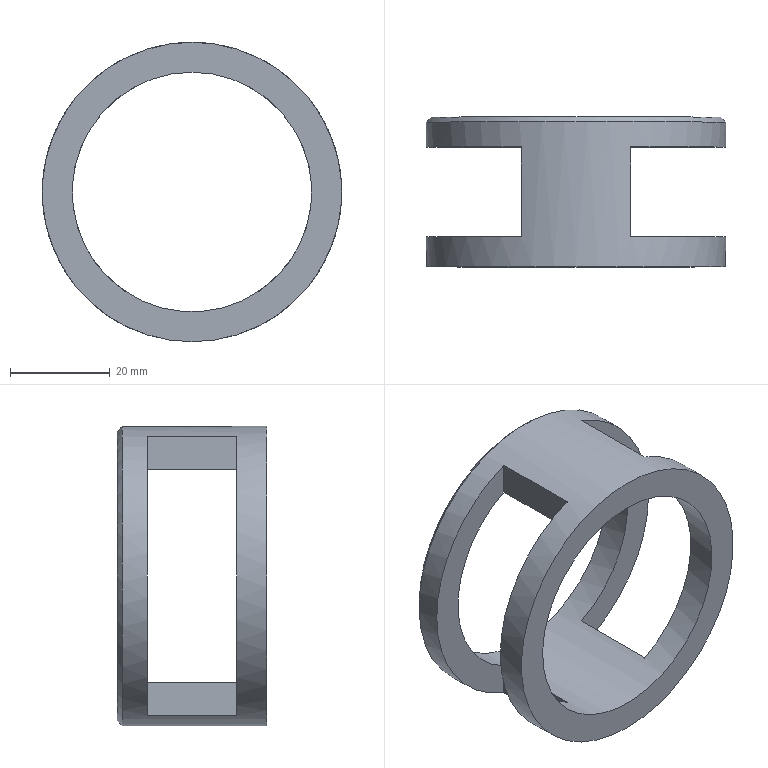Component | NX | BUSHING | 1 solid | 13 faces | box 60 x 30 x 60 mm | volume 17018 mm3 | plane 10 | cylinder 2 | cone 1 | commonest cylinder face diameters 60 x1 48 x1
STEP:
#1=CARTESIAN_POINT('',(0.,0.,0.));
#2=DIRECTION('',(0.,0.,1.));
#3=DIRECTION('',(1.,0.,0.));
#4=AXIS2_PLACEMENT_3D('',#1,#2,#3);
#5=CARTESIAN_POINT('',(-0.,-5.,-25.5));
#6=VERTEX_POINT('',#5);
#7=CARTESIAN_POINT('',(-0.,-5.,4.5));
#8=DIRECTION('',(0.,-1.,0.));
#9=DIRECTION('',(0.,0.,-1.));
#10=AXIS2_PLACEMENT_3D('',#7,#8,#9);
#11=CIRCLE('',#10,30.);
#12=CARTESIAN_POINT('',(-0.,-34.,4.5));
#13=DIRECTION('',(0.,1.,0.));
#14=DIRECTION('',(0.,0.,-1.));
#15=AXIS2_PLACEMENT_3D('',#12,#13,#14);
#16=CYLINDRICAL_SURFACE('',#15,30.);
#17=CARTESIAN_POINT('',(6.283,29.));
#18=DIRECTION('',(-1.,0.));
#19=VECTOR('',#18,1.);
#20=LINE('',#17,#19);
#21=(GEOMETRIC_REPRESENTATION_CONTEXT(2)PARAMETRIC_REPRESENTATION_CONTEXT()REPRESENTATION_CONTEXT('',''));
#22=DEFINITIONAL_REPRESENTATION('',(#20),#21);
#23=PCURVE('',#16,#22);
#24=CARTESIAN_POINT('',(-0.,-4.,4.5));
#25=DIRECTION('',(0.,-1.,0.));
#26=DIRECTION('',(0.,0.,1.));
#27=AXIS2_PLACEMENT_3D('',#24,#25,#26);
#28=CONICAL_SURFACE('',#27,29.,0.7854);
#29=CARTESIAN_POINT('',(3.142,1.));
#30=DIRECTION('',(1.,0.));
#31=VECTOR('',#30,1.);
#32=LINE('',#29,#31);
#33=(GEOMETRIC_REPRESENTATION_CONTEXT(2)PARAMETRIC_REPRESENTATION_CONTEXT()REPRESENTATION_CONTEXT('',''));
#34=DEFINITIONAL_REPRESENTATION('',(#32),#33);
#35=PCURVE('',#28,#34);
#36=SURFACE_CURVE('',#11,(#23,#35),.PCURVE_S1.);
#37=EDGE_CURVE('',#6,#6,#36,.T.);
#38=ORIENTED_EDGE('',*,*,#37,.T.);
#39=CARTESIAN_POINT('',(0.,-34.,-25.5));
#40=VERTEX_POINT('',#39);
#41=CARTESIAN_POINT('',(0.,-34.,-25.5));
#42=CARTESIAN_POINT('',(0.,-5.,-25.5));
#43=B_SPLINE_CURVE_WITH_KNOTS('',1,(#41,#42),.UNSPECIFIED.,.F.,.F.,(2,2),(0.,29.),.PIECEWISE_BEZIER_KNOTS.);
#44=CARTESIAN_POINT('',(0.,0.));
#45=DIRECTION('',(0.,1.));
#46=VECTOR('',#45,1.);
#47=LINE('',#44,#46);
#48=(GEOMETRIC_REPRESENTATION_CONTEXT(2)PARAMETRIC_REPRESENTATION_CONTEXT()REPRESENTATION_CONTEXT('',''));
#49=DEFINITIONAL_REPRESENTATION('',(#47),#48);
#50=PCURVE('',#16,#49);
#51=CARTESIAN_POINT('',(6.283,0.));
#52=DIRECTION('',(0.,1.));
#53=VECTOR('',#52,1.);
#54=LINE('',#51,#53);
#55=(GEOMETRIC_REPRESENTATION_CONTEXT(2)PARAMETRIC_REPRESENTATION_CONTEXT()REPRESENTATION_CONTEXT('',''));
#56=DEFINITIONAL_REPRESENTATION('',(#54),#55);
#57=PCURVE('',#16,#56);
#58=SEAM_CURVE('',#43,(#50,#57),.PCURVE_S1.);
#59=EDGE_CURVE('',#40,#6,#58,.T.);
#60=ORIENTED_EDGE('',*,*,#59,.F.);
#61=CARTESIAN_POINT('',(-0.,-34.,34.5));
#62=VERTEX_POINT('',#61);
#63=CARTESIAN_POINT('',(-0.,-34.,4.5));
#64=DIRECTION('',(0.,1.,0.));
#65=DIRECTION('',(-0.,0.,1.));
#66=AXIS2_PLACEMENT_3D('',#63,#64,#65);
#67=CIRCLE('',#66,30.);
#68=CARTESIAN_POINT('',(-3.142,0.));
#69=DIRECTION('',(1.,0.));
#70=VECTOR('',#69,1.);
#71=LINE('',#68,#70);
#72=(GEOMETRIC_REPRESENTATION_CONTEXT(2)PARAMETRIC_REPRESENTATION_CONTEXT()REPRESENTATION_CONTEXT('',''));
#73=DEFINITIONAL_REPRESENTATION('',(#71),#72);
#74=PCURVE('',#16,#73);
#75=CARTESIAN_POINT('',(-0.,-34.,4.5));
#76=DIRECTION('',(0.,1.,0.));
#77=DIRECTION('',(0.,0.,-1.));
#78=AXIS2_PLACEMENT_3D('',#75,#76,#77);
#79=PLANE('',#78);
#80=CARTESIAN_POINT('',(0.,0.));
#81=DIRECTION('',(-1.,0.));
#82=AXIS2_PLACEMENT_2D('',#80,#81);
#83=CIRCLE('',#82,30.);
#84=(GEOMETRIC_REPRESENTATION_CONTEXT(2)PARAMETRIC_REPRESENTATION_CONTEXT()REPRESENTATION_CONTEXT('',''));
#85=DEFINITIONAL_REPRESENTATION('',(#83),#84);
#86=PCURVE('',#79,#85);
#87=SURFACE_CURVE('',#67,(#74,#86),.PCURVE_S1.);
#88=EDGE_CURVE('',#40,#62,#87,.T.);
#89=ORIENTED_EDGE('',*,*,#88,.T.);
#90=CARTESIAN_POINT('',(-0.,-34.,4.5));
#91=DIRECTION('',(0.,1.,0.));
#92=DIRECTION('',(-0.,0.,1.));
#93=AXIS2_PLACEMENT_3D('',#90,#91,#92);
#94=CIRCLE('',#93,30.);
#95=CARTESIAN_POINT('',(3.142,0.));
#96=DIRECTION('',(1.,0.));
#97=VECTOR('',#96,1.);
#98=LINE('',#95,#97);
#99=(GEOMETRIC_REPRESENTATION_CONTEXT(2)PARAMETRIC_REPRESENTATION_CONTEXT()REPRESENTATION_CONTEXT('',''));
#100=DEFINITIONAL_REPRESENTATION('',(#98),#99);
#101=PCURVE('',#16,#100);
#102=CARTESIAN_POINT('',(0.,0.));
#103=DIRECTION('',(-1.,0.));
#104=AXIS2_PLACEMENT_2D('',#102,#103);
#105=CIRCLE('',#104,30.);
#106=(GEOMETRIC_REPRESENTATION_CONTEXT(2)PARAMETRIC_REPRESENTATION_CONTEXT()REPRESENTATION_CONTEXT('',''));
#107=DEFINITIONAL_REPRESENTATION('',(#105),#106);
#108=PCURVE('',#79,#107);
#109=SURFACE_CURVE('',#94,(#101,#108),.PCURVE_S1.);
#110=EDGE_CURVE('',#62,#40,#109,.T.);
#111=ORIENTED_EDGE('',*,*,#110,.T.);
#112=ORIENTED_EDGE('',*,*,#59,.T.);
#113=EDGE_LOOP('',(#38,#60,#89,#111,#112));
#114=FACE_BOUND('',#113,.T.);
#115=CARTESIAN_POINT('',(11.,-28.,32.411));
#116=VERTEX_POINT('',#115);
#117=CARTESIAN_POINT('',(11.,-28.,-23.411));
#118=VERTEX_POINT('',#117);
#119=CARTESIAN_POINT('',(-0.,-28.,4.5));
#120=DIRECTION('',(0.,1.,0.));
#121=DIRECTION('',(0.,0.,1.));
#122=AXIS2_PLACEMENT_3D('',#119,#120,#121);
#123=CIRCLE('',#122,30.);
#124=CARTESIAN_POINT('',(3.142,6.));
#125=DIRECTION('',(1.,0.));
#126=VECTOR('',#125,1.);
#127=LINE('',#124,#126);
#128=(GEOMETRIC_REPRESENTATION_CONTEXT(2)PARAMETRIC_REPRESENTATION_CONTEXT()REPRESENTATION_CONTEXT('',''));
#129=DEFINITIONAL_REPRESENTATION('',(#127),#128);
#130=PCURVE('',#16,#129);
#131=CARTESIAN_POINT('',(36.,-28.,54.5));
#132=DIRECTION('',(0.,-1.,0.));
#133=DIRECTION('',(0.,0.,1.));
#134=AXIS2_PLACEMENT_3D('',#131,#132,#133);
#135=PLANE('',#134);
#136=CARTESIAN_POINT('',(-20.,36.));
#137=CARTESIAN_POINT('',(-20.,-15.962));
#138=CARTESIAN_POINT('',(-65.,10.019));
#139=CARTESIAN_POINT('',(-110.,36.));
#140=CARTESIAN_POINT('',(-65.,61.981));
#141=CARTESIAN_POINT('',(-20.,87.962));
#142=CARTESIAN_POINT('',(-20.,36.));
#143=(BOUNDED_CURVE()B_SPLINE_CURVE(2,(#136,#137,#138,#139,#140,#141,#142),.UNSPECIFIED.,.T.,.F.)B_SPLINE_CURVE_WITH_KNOTS((1,2,2,2,2,1),(-2.094,0.,2.094,4.189,6.283,8.378),.UNSPECIFIED.)CURVE()GEOMETRIC_REPRESENTATION_ITEM()RATIONAL_B_SPLINE_CURVE((1.,0.5,1.,0.5,1.,0.5,1.))REPRESENTATION_ITEM(''));
#144=(GEOMETRIC_REPRESENTATION_CONTEXT(2)PARAMETRIC_REPRESENTATION_CONTEXT()REPRESENTATION_CONTEXT('',''));
#145=DEFINITIONAL_REPRESENTATION('',(#143),#144);
#146=PCURVE('',#135,#145);
#147=SURFACE_CURVE('',#123,(#130,#146),.PCURVE_S1.);
#148=EDGE_CURVE('',#116,#118,#147,.T.);
#149=ORIENTED_EDGE('',*,*,#148,.F.);
#150=CARTESIAN_POINT('',(11.,-10.,32.411));
#151=VERTEX_POINT('',#150);
#152=CARTESIAN_POINT('',(11.,-34.,32.411));
#153=DIRECTION('',(0.,-1.,0.));
#154=VECTOR('',#153,1.);
#155=LINE('',#152,#154);
#156=CARTESIAN_POINT('',(3.517,0.));
#157=DIRECTION('',(0.,-1.));
#158=VECTOR('',#157,1.);
#159=LINE('',#156,#158);
#160=(GEOMETRIC_REPRESENTATION_CONTEXT(2)PARAMETRIC_REPRESENTATION_CONTEXT()REPRESENTATION_CONTEXT('',''));
#161=DEFINITIONAL_REPRESENTATION('',(#159),#160);
#162=PCURVE('',#16,#161);
#163=CARTESIAN_POINT('',(11.,-28.,54.5));
#164=DIRECTION('',(-1.,-0.,0.));
#165=DIRECTION('',(0.,-1.,0.));
#166=AXIS2_PLACEMENT_3D('',#163,#164,#165);
#167=PLANE('',#166);
#168=CARTESIAN_POINT('',(6.,-22.089));
#169=DIRECTION('',(1.,0.));
#170=VECTOR('',#169,1.);
#171=LINE('',#168,#170);
#172=(GEOMETRIC_REPRESENTATION_CONTEXT(2)PARAMETRIC_REPRESENTATION_CONTEXT()REPRESENTATION_CONTEXT('',''));
#173=DEFINITIONAL_REPRESENTATION('',(#171),#172);
#174=PCURVE('',#167,#173);
#175=SURFACE_CURVE('',#155,(#162,#174),.PCURVE_S1.);
#176=EDGE_CURVE('',#151,#116,#175,.T.);
#177=ORIENTED_EDGE('',*,*,#176,.F.);
#178=CARTESIAN_POINT('',(11.,-10.,-23.411));
#179=VERTEX_POINT('',#178);
#180=CARTESIAN_POINT('',(-0.,-10.,4.5));
#181=DIRECTION('',(0.,-1.,0.));
#182=DIRECTION('',(-1.,-0.,0.));
#183=AXIS2_PLACEMENT_3D('',#180,#181,#182);
#184=CIRCLE('',#183,30.);
#185=CARTESIAN_POINT('',(7.854,24.));
#186=DIRECTION('',(-1.,0.));
#187=VECTOR('',#186,1.);
#188=LINE('',#185,#187);
#189=(GEOMETRIC_REPRESENTATION_CONTEXT(2)PARAMETRIC_REPRESENTATION_CONTEXT()REPRESENTATION_CONTEXT('',''));
#190=DEFINITIONAL_REPRESENTATION('',(#188),#189);
#191=PCURVE('',#16,#190);
#192=CARTESIAN_POINT('',(11.,-10.,54.5));
#193=DIRECTION('',(-0.,1.,0.));
#194=DIRECTION('',(-1.,-0.,0.));
#195=AXIS2_PLACEMENT_3D('',#192,#193,#194);
#196=PLANE('',#195);
#197=CARTESIAN_POINT('',(41.,-50.));
#198=CARTESIAN_POINT('',(41.,-101.962));
#199=CARTESIAN_POINT('',(-4.,-75.981));
#200=CARTESIAN_POINT('',(-49.,-50.));
#201=CARTESIAN_POINT('',(-4.,-24.019));
#202=CARTESIAN_POINT('',(41.,1.962));
#203=CARTESIAN_POINT('',(41.,-50.));
#204=(BOUNDED_CURVE()B_SPLINE_CURVE(2,(#197,#198,#199,#200,#201,#202,#203),.UNSPECIFIED.,.T.,.F.)B_SPLINE_CURVE_WITH_KNOTS((1,2,2,2,2,1),(-2.094,0.,2.094,4.189,6.283,8.378),.UNSPECIFIED.)CURVE()GEOMETRIC_REPRESENTATION_ITEM()RATIONAL_B_SPLINE_CURVE((1.,0.5,1.,0.5,1.,0.5,1.))REPRESENTATION_ITEM(''));
#205=(GEOMETRIC_REPRESENTATION_CONTEXT(2)PARAMETRIC_REPRESENTATION_CONTEXT()REPRESENTATION_CONTEXT('',''));
#206=DEFINITIONAL_REPRESENTATION('',(#204),#205);
#207=PCURVE('',#196,#206);
#208=SURFACE_CURVE('',#184,(#191,#207),.PCURVE_S1.);
#209=EDGE_CURVE('',#179,#151,#208,.T.);
#210=ORIENTED_EDGE('',*,*,#209,.F.);
#211=CARTESIAN_POINT('',(11.,-34.,-23.411));
#212=DIRECTION('',(0.,1.,0.));
#213=VECTOR('',#212,1.);
#214=LINE('',#211,#213);
#215=CARTESIAN_POINT('',(5.908,0.));
#216=DIRECTION('',(0.,1.));
#217=VECTOR('',#216,1.);
#218=LINE('',#215,#217);
#219=(GEOMETRIC_REPRESENTATION_CONTEXT(2)PARAMETRIC_REPRESENTATION_CONTEXT()REPRESENTATION_CONTEXT('',''));
#220=DEFINITIONAL_REPRESENTATION('',(#218),#219);
#221=PCURVE('',#16,#220);
#222=CARTESIAN_POINT('',(11.,-28.,54.5));
#223=DIRECTION('',(-1.,-0.,0.));
#224=DIRECTION('',(0.,-1.,0.));
#225=AXIS2_PLACEMENT_3D('',#222,#223,#224);
#226=PLANE('',#225);
#227=CARTESIAN_POINT('',(6.,-77.911));
#228=DIRECTION('',(-1.,0.));
#229=VECTOR('',#228,1.);
#230=LINE('',#227,#229);
#231=(GEOMETRIC_REPRESENTATION_CONTEXT(2)PARAMETRIC_REPRESENTATION_CONTEXT()REPRESENTATION_CONTEXT('',''));
#232=DEFINITIONAL_REPRESENTATION('',(#230),#231);
#233=PCURVE('',#226,#232);
#234=SURFACE_CURVE('',#214,(#221,#233),.PCURVE_S1.);
#235=EDGE_CURVE('',#118,#179,#234,.T.);
#236=ORIENTED_EDGE('',*,*,#235,.F.);
#237=EDGE_LOOP('',(#149,#177,#210,#236));
#238=FACE_BOUND('',#237,.T.);
#239=CARTESIAN_POINT('',(-11.,-28.,-23.411));
#240=VERTEX_POINT('',#239);
#241=CARTESIAN_POINT('',(-11.,-10.,-23.411));
#242=VERTEX_POINT('',#241);
#243=CARTESIAN_POINT('',(-11.,-34.,-23.411));
#244=DIRECTION('',(0.,1.,0.));
#245=VECTOR('',#244,1.);
#246=LINE('',#243,#245);
#247=CARTESIAN_POINT('',(0.3754,0.));
#248=DIRECTION('',(0.,1.));
#249=VECTOR('',#248,1.);
#250=LINE('',#247,#249);
#251=(GEOMETRIC_REPRESENTATION_CONTEXT(2)PARAMETRIC_REPRESENTATION_CONTEXT()REPRESENTATION_CONTEXT('',''));
#252=DEFINITIONAL_REPRESENTATION('',(#250),#251);
#253=PCURVE('',#16,#252);
#254=CARTESIAN_POINT('',(-11.,-28.,54.5));
#255=DIRECTION('',(-1.,0.,0.));
#256=DIRECTION('',(-0.,-1.,0.));
#257=AXIS2_PLACEMENT_3D('',#254,#255,#256);
#258=PLANE('',#257);
#259=CARTESIAN_POINT('',(6.,-77.911));
#260=DIRECTION('',(-1.,0.));
#261=VECTOR('',#260,1.);
#262=LINE('',#259,#261);
#263=(GEOMETRIC_REPRESENTATION_CONTEXT(2)PARAMETRIC_REPRESENTATION_CONTEXT()REPRESENTATION_CONTEXT('',''));
#264=DEFINITIONAL_REPRESENTATION('',(#262),#263);
#265=PCURVE('',#258,#264);
#266=SURFACE_CURVE('',#246,(#253,#265),.PCURVE_S1.);
#267=EDGE_CURVE('',#240,#242,#266,.T.);
#268=ORIENTED_EDGE('',*,*,#267,.T.);
#269=CARTESIAN_POINT('',(-11.,-10.,32.411));
#270=VERTEX_POINT('',#269);
#271=CARTESIAN_POINT('',(-0.,-10.,4.5));
#272=DIRECTION('',(0.,1.,0.));
#273=DIRECTION('',(1.,-0.,0.));
#274=AXIS2_PLACEMENT_3D('',#271,#272,#273);
#275=CIRCLE('',#274,30.);
#276=CARTESIAN_POINT('',(-1.571,24.));
#277=DIRECTION('',(1.,0.));
#278=VECTOR('',#277,1.);
#279=LINE('',#276,#278);
#280=(GEOMETRIC_REPRESENTATION_CONTEXT(2)PARAMETRIC_REPRESENTATION_CONTEXT()REPRESENTATION_CONTEXT('',''));
#281=DEFINITIONAL_REPRESENTATION('',(#279),#280);
#282=PCURVE('',#16,#281);
#283=CARTESIAN_POINT('',(-11.,-10.,54.5));
#284=DIRECTION('',(-0.,-1.,0.));
#285=DIRECTION('',(1.,-0.,0.));
#286=AXIS2_PLACEMENT_3D('',#283,#284,#285);
#287=PLANE('',#286);
#288=CARTESIAN_POINT('',(41.,-50.));
#289=CARTESIAN_POINT('',(41.,-101.962));
#290=CARTESIAN_POINT('',(-4.,-75.981));
#291=CARTESIAN_POINT('',(-49.,-50.));
#292=CARTESIAN_POINT('',(-4.,-24.019));
#293=CARTESIAN_POINT('',(41.,1.962));
#294=CARTESIAN_POINT('',(41.,-50.));
#295=(BOUNDED_CURVE()B_SPLINE_CURVE(2,(#288,#289,#290,#291,#292,#293,#294),.UNSPECIFIED.,.T.,.F.)B_SPLINE_CURVE_WITH_KNOTS((1,2,2,2,2,1),(-2.094,0.,2.094,4.189,6.283,8.378),.UNSPECIFIED.)CURVE()GEOMETRIC_REPRESENTATION_ITEM()RATIONAL_B_SPLINE_CURVE((1.,0.5,1.,0.5,1.,0.5,1.))REPRESENTATION_ITEM(''));
#296=(GEOMETRIC_REPRESENTATION_CONTEXT(2)PARAMETRIC_REPRESENTATION_CONTEXT()REPRESENTATION_CONTEXT('',''));
#297=DEFINITIONAL_REPRESENTATION('',(#295),#296);
#298=PCURVE('',#287,#297);
#299=SURFACE_CURVE('',#275,(#282,#298),.PCURVE_S1.);
#300=EDGE_CURVE('',#242,#270,#299,.T.);
#301=ORIENTED_EDGE('',*,*,#300,.T.);
#302=CARTESIAN_POINT('',(-11.,-28.,32.411));
#303=VERTEX_POINT('',#302);
#304=CARTESIAN_POINT('',(-11.,-34.,32.411));
#305=DIRECTION('',(0.,-1.,0.));
#306=VECTOR('',#305,1.);
#307=LINE('',#304,#306);
#308=CARTESIAN_POINT('',(2.766,0.));
#309=DIRECTION('',(0.,-1.));
#310=VECTOR('',#309,1.);
#311=LINE('',#308,#310);
#312=(GEOMETRIC_REPRESENTATION_CONTEXT(2)PARAMETRIC_REPRESENTATION_CONTEXT()REPRESENTATION_CONTEXT('',''));
#313=DEFINITIONAL_REPRESENTATION('',(#311),#312);
#314=PCURVE('',#16,#313);
#315=CARTESIAN_POINT('',(-11.,-28.,54.5));
#316=DIRECTION('',(-1.,0.,0.));
#317=DIRECTION('',(-0.,-1.,0.));
#318=AXIS2_PLACEMENT_3D('',#315,#316,#317);
#319=PLANE('',#318);
#320=CARTESIAN_POINT('',(6.,-22.089));
#321=DIRECTION('',(1.,0.));
#322=VECTOR('',#321,1.);
#323=LINE('',#320,#322);
#324=(GEOMETRIC_REPRESENTATION_CONTEXT(2)PARAMETRIC_REPRESENTATION_CONTEXT()REPRESENTATION_CONTEXT('',''));
#325=DEFINITIONAL_REPRESENTATION('',(#323),#324);
#326=PCURVE('',#319,#325);
#327=SURFACE_CURVE('',#307,(#314,#326),.PCURVE_S1.);
#328=EDGE_CURVE('',#270,#303,#327,.T.);
#329=ORIENTED_EDGE('',*,*,#328,.T.);
#330=CARTESIAN_POINT('',(-0.,-28.,4.5));
#331=DIRECTION('',(0.,-1.,0.));
#332=DIRECTION('',(0.,0.,-1.));
#333=AXIS2_PLACEMENT_3D('',#330,#331,#332);
#334=CIRCLE('',#333,30.);
#335=CARTESIAN_POINT('',(6.283,6.));
#336=DIRECTION('',(-1.,0.));
#337=VECTOR('',#336,1.);
#338=LINE('',#335,#337);
#339=(GEOMETRIC_REPRESENTATION_CONTEXT(2)PARAMETRIC_REPRESENTATION_CONTEXT()REPRESENTATION_CONTEXT('',''));
#340=DEFINITIONAL_REPRESENTATION('',(#338),#339);
#341=PCURVE('',#16,#340);
#342=CARTESIAN_POINT('',(-36.,-28.,54.5));
#343=DIRECTION('',(0.,1.,0.));
#344=DIRECTION('',(0.,0.,-1.));
#345=AXIS2_PLACEMENT_3D('',#342,#343,#344);
#346=PLANE('',#345);
#347=CARTESIAN_POINT('',(80.,-36.));
#348=CARTESIAN_POINT('',(80.,-87.962));
#349=CARTESIAN_POINT('',(35.,-61.981));
#350=CARTESIAN_POINT('',(-10.,-36.));
#351=CARTESIAN_POINT('',(35.,-10.019));
#352=CARTESIAN_POINT('',(80.,15.962));
#353=CARTESIAN_POINT('',(80.,-36.));
#354=(BOUNDED_CURVE()B_SPLINE_CURVE(2,(#347,#348,#349,#350,#351,#352,#353),.UNSPECIFIED.,.T.,.F.)B_SPLINE_CURVE_WITH_KNOTS((1,2,2,2,2,1),(-2.094,0.,2.094,4.189,6.283,8.378),.UNSPECIFIED.)CURVE()GEOMETRIC_REPRESENTATION_ITEM()RATIONAL_B_SPLINE_CURVE((1.,0.5,1.,0.5,1.,0.5,1.))REPRESENTATION_ITEM(''));
#355=(GEOMETRIC_REPRESENTATION_CONTEXT(2)PARAMETRIC_REPRESENTATION_CONTEXT()REPRESENTATION_CONTEXT('',''));
#356=DEFINITIONAL_REPRESENTATION('',(#354),#355);
#357=PCURVE('',#346,#356);
#358=SURFACE_CURVE('',#334,(#341,#357),.PCURVE_S1.);
#359=EDGE_CURVE('',#303,#240,#358,.T.);
#360=ORIENTED_EDGE('',*,*,#359,.T.);
#361=EDGE_LOOP('',(#268,#301,#329,#360));
#362=FACE_BOUND('',#361,.T.);
#363=ADVANCED_FACE('',(#114,#238,#362),#16,.T.);
#364=CARTESIAN_POINT('',(-0.,-4.,28.5));
#365=VERTEX_POINT('',#364);
#366=CARTESIAN_POINT('',(-0.,-4.,4.5));
#367=DIRECTION('',(0.,1.,0.));
#368=DIRECTION('',(-0.,0.,1.));
#369=AXIS2_PLACEMENT_3D('',#366,#367,#368);
#370=CIRCLE('',#369,24.);
#371=CARTESIAN_POINT('',(-0.,-34.,4.5));
#372=DIRECTION('',(0.,1.,0.));
#373=DIRECTION('',(0.,0.,-1.));
#374=AXIS2_PLACEMENT_3D('',#371,#372,#373);
#375=CYLINDRICAL_SURFACE('',#374,24.);
#376=CARTESIAN_POINT('',(3.142,30.));
#377=DIRECTION('',(1.,0.));
#378=VECTOR('',#377,1.);
#379=LINE('',#376,#378);
#380=(GEOMETRIC_REPRESENTATION_CONTEXT(2)PARAMETRIC_REPRESENTATION_CONTEXT()REPRESENTATION_CONTEXT('',''));
#381=DEFINITIONAL_REPRESENTATION('',(#379),#380);
#382=PCURVE('',#375,#381);
#383=CARTESIAN_POINT('',(-0.,-4.,4.5));
#384=DIRECTION('',(0.,1.,0.));
#385=DIRECTION('',(0.,0.,-1.));
#386=AXIS2_PLACEMENT_3D('',#383,#384,#385);
#387=PLANE('',#386);
#388=CARTESIAN_POINT('',(0.,0.));
#389=DIRECTION('',(-1.,0.));
#390=AXIS2_PLACEMENT_2D('',#388,#389);
#391=CIRCLE('',#390,24.);
#392=(GEOMETRIC_REPRESENTATION_CONTEXT(2)PARAMETRIC_REPRESENTATION_CONTEXT()REPRESENTATION_CONTEXT('',''));
#393=DEFINITIONAL_REPRESENTATION('',(#391),#392);
#394=PCURVE('',#387,#393);
#395=SURFACE_CURVE('',#370,(#382,#394),.PCURVE_S1.);
#396=EDGE_CURVE('',#365,#365,#395,.T.);
#397=ORIENTED_EDGE('',*,*,#396,.F.);
#398=CARTESIAN_POINT('',(-0.,-34.,28.5));
#399=VERTEX_POINT('',#398);
#400=CARTESIAN_POINT('',(-0.,-34.,28.5));
#401=CARTESIAN_POINT('',(-0.,-4.,28.5));
#402=B_SPLINE_CURVE_WITH_KNOTS('',1,(#400,#401),.UNSPECIFIED.,.F.,.F.,(2,2),(0.,30.),.PIECEWISE_BEZIER_KNOTS.);
#403=CARTESIAN_POINT('',(3.142,0.));
#404=DIRECTION('',(0.,1.));
#405=VECTOR('',#404,1.);
#406=LINE('',#403,#405);
#407=(GEOMETRIC_REPRESENTATION_CONTEXT(2)PARAMETRIC_REPRESENTATION_CONTEXT()REPRESENTATION_CONTEXT('',''));
#408=DEFINITIONAL_REPRESENTATION('',(#406),#407);
#409=PCURVE('',#375,#408);
#410=CARTESIAN_POINT('',(9.425,0.));
#411=DIRECTION('',(0.,1.));
#412=VECTOR('',#411,1.);
#413=LINE('',#410,#412);
#414=(GEOMETRIC_REPRESENTATION_CONTEXT(2)PARAMETRIC_REPRESENTATION_CONTEXT()REPRESENTATION_CONTEXT('',''));
#415=DEFINITIONAL_REPRESENTATION('',(#413),#414);
#416=PCURVE('',#375,#415);
#417=SEAM_CURVE('',#402,(#409,#416),.PCURVE_S1.);
#418=EDGE_CURVE('',#399,#365,#417,.T.);
#419=ORIENTED_EDGE('',*,*,#418,.F.);
#420=CARTESIAN_POINT('',(-0.,-34.,4.5));
#421=DIRECTION('',(0.,1.,0.));
#422=DIRECTION('',(-0.,0.,1.));
#423=AXIS2_PLACEMENT_3D('',#420,#421,#422);
#424=CIRCLE('',#423,24.);
#425=CARTESIAN_POINT('',(3.142,0.));
#426=DIRECTION('',(1.,0.));
#427=VECTOR('',#426,1.);
#428=LINE('',#425,#427);
#429=(GEOMETRIC_REPRESENTATION_CONTEXT(2)PARAMETRIC_REPRESENTATION_CONTEXT()REPRESENTATION_CONTEXT('',''));
#430=DEFINITIONAL_REPRESENTATION('',(#428),#429);
#431=PCURVE('',#375,#430);
#432=CARTESIAN_POINT('',(0.,0.));
#433=DIRECTION('',(-1.,0.));
#434=AXIS2_PLACEMENT_2D('',#432,#433);
#435=CIRCLE('',#434,24.);
#436=(GEOMETRIC_REPRESENTATION_CONTEXT(2)PARAMETRIC_REPRESENTATION_CONTEXT()REPRESENTATION_CONTEXT('',''));
#437=DEFINITIONAL_REPRESENTATION('',(#435),#436);
#438=PCURVE('',#79,#437);
#439=SURFACE_CURVE('',#424,(#431,#438),.PCURVE_S1.);
#440=EDGE_CURVE('',#399,#399,#439,.T.);
#441=ORIENTED_EDGE('',*,*,#440,.T.);
#442=ORIENTED_EDGE('',*,*,#418,.T.);
#443=EDGE_LOOP('',(#397,#419,#441,#442));
#444=FACE_BOUND('',#443,.F.);
#445=CARTESIAN_POINT('',(11.,-10.,-16.831));
#446=VERTEX_POINT('',#445);
#447=CARTESIAN_POINT('',(11.,-10.,25.831));
#448=VERTEX_POINT('',#447);
#449=CARTESIAN_POINT('',(-0.,-10.,4.5));
#450=DIRECTION('',(0.,-1.,0.));
#451=DIRECTION('',(-1.,-0.,0.));
#452=AXIS2_PLACEMENT_3D('',#449,#450,#451);
#453=CIRCLE('',#452,24.);
#454=CARTESIAN_POINT('',(7.854,24.));
#455=DIRECTION('',(-1.,0.));
#456=VECTOR('',#455,1.);
#457=LINE('',#454,#456);
#458=(GEOMETRIC_REPRESENTATION_CONTEXT(2)PARAMETRIC_REPRESENTATION_CONTEXT()REPRESENTATION_CONTEXT('',''));
#459=DEFINITIONAL_REPRESENTATION('',(#457),#458);
#460=PCURVE('',#375,#459);
#461=CARTESIAN_POINT('',(35.,-50.));
#462=CARTESIAN_POINT('',(35.,-91.569));
#463=CARTESIAN_POINT('',(-1.,-70.785));
#464=CARTESIAN_POINT('',(-37.,-50.));
#465=CARTESIAN_POINT('',(-1.,-29.215));
#466=CARTESIAN_POINT('',(35.,-8.431));
#467=CARTESIAN_POINT('',(35.,-50.));
#468=(BOUNDED_CURVE()B_SPLINE_CURVE(2,(#461,#462,#463,#464,#465,#466,#467),.UNSPECIFIED.,.T.,.F.)B_SPLINE_CURVE_WITH_KNOTS((1,2,2,2,2,1),(-2.094,0.,2.094,4.189,6.283,8.378),.UNSPECIFIED.)CURVE()GEOMETRIC_REPRESENTATION_ITEM()RATIONAL_B_SPLINE_CURVE((1.,0.5,1.,0.5,1.,0.5,1.))REPRESENTATION_ITEM(''));
#469=(GEOMETRIC_REPRESENTATION_CONTEXT(2)PARAMETRIC_REPRESENTATION_CONTEXT()REPRESENTATION_CONTEXT('',''));
#470=DEFINITIONAL_REPRESENTATION('',(#468),#469);
#471=PCURVE('',#196,#470);
#472=SURFACE_CURVE('',#453,(#460,#471),.PCURVE_S1.);
#473=EDGE_CURVE('',#446,#448,#472,.T.);
#474=ORIENTED_EDGE('',*,*,#473,.F.);
#475=CARTESIAN_POINT('',(11.,-28.,-16.831));
#476=VERTEX_POINT('',#475);
#477=CARTESIAN_POINT('',(11.,-34.,-16.831));
#478=DIRECTION('',(0.,1.,0.));
#479=VECTOR('',#478,1.);
#480=LINE('',#477,#479);
#481=CARTESIAN_POINT('',(5.807,0.));
#482=DIRECTION('',(0.,1.));
#483=VECTOR('',#482,1.);
#484=LINE('',#481,#483);
#485=(GEOMETRIC_REPRESENTATION_CONTEXT(2)PARAMETRIC_REPRESENTATION_CONTEXT()REPRESENTATION_CONTEXT('',''));
#486=DEFINITIONAL_REPRESENTATION('',(#484),#485);
#487=PCURVE('',#375,#486);
#488=CARTESIAN_POINT('',(6.,-71.331));
#489=DIRECTION('',(-1.,0.));
#490=VECTOR('',#489,1.);
#491=LINE('',#488,#490);
#492=(GEOMETRIC_REPRESENTATION_CONTEXT(2)PARAMETRIC_REPRESENTATION_CONTEXT()REPRESENTATION_CONTEXT('',''));
#493=DEFINITIONAL_REPRESENTATION('',(#491),#492);
#494=PCURVE('',#226,#493);
#495=SURFACE_CURVE('',#480,(#487,#494),.PCURVE_S1.);
#496=EDGE_CURVE('',#476,#446,#495,.T.);
#497=ORIENTED_EDGE('',*,*,#496,.F.);
#498=CARTESIAN_POINT('',(11.,-28.,25.831));
#499=VERTEX_POINT('',#498);
#500=CARTESIAN_POINT('',(-0.,-28.,4.5));
#501=DIRECTION('',(0.,1.,0.));
#502=DIRECTION('',(0.,0.,1.));
#503=AXIS2_PLACEMENT_3D('',#500,#501,#502);
#504=CIRCLE('',#503,24.);
#505=CARTESIAN_POINT('',(3.142,6.));
#506=DIRECTION('',(1.,0.));
#507=VECTOR('',#506,1.);
#508=LINE('',#505,#507);
#509=(GEOMETRIC_REPRESENTATION_CONTEXT(2)PARAMETRIC_REPRESENTATION_CONTEXT()REPRESENTATION_CONTEXT('',''));
#510=DEFINITIONAL_REPRESENTATION('',(#508),#509);
#511=PCURVE('',#375,#510);
#512=CARTESIAN_POINT('',(-26.,36.));
#513=CARTESIAN_POINT('',(-26.,-5.569));
#514=CARTESIAN_POINT('',(-62.,15.215));
#515=CARTESIAN_POINT('',(-98.,36.));
#516=CARTESIAN_POINT('',(-62.,56.785));
#517=CARTESIAN_POINT('',(-26.,77.569));
#518=CARTESIAN_POINT('',(-26.,36.));
#519=(BOUNDED_CURVE()B_SPLINE_CURVE(2,(#512,#513,#514,#515,#516,#517,#518),.UNSPECIFIED.,.T.,.F.)B_SPLINE_CURVE_WITH_KNOTS((1,2,2,2,2,1),(-2.094,0.,2.094,4.189,6.283,8.378),.UNSPECIFIED.)CURVE()GEOMETRIC_REPRESENTATION_ITEM()RATIONAL_B_SPLINE_CURVE((1.,0.5,1.,0.5,1.,0.5,1.))REPRESENTATION_ITEM(''));
#520=(GEOMETRIC_REPRESENTATION_CONTEXT(2)PARAMETRIC_REPRESENTATION_CONTEXT()REPRESENTATION_CONTEXT('',''));
#521=DEFINITIONAL_REPRESENTATION('',(#519),#520);
#522=PCURVE('',#135,#521);
#523=SURFACE_CURVE('',#504,(#511,#522),.PCURVE_S1.);
#524=EDGE_CURVE('',#499,#476,#523,.T.);
#525=ORIENTED_EDGE('',*,*,#524,.F.);
#526=CARTESIAN_POINT('',(11.,-34.,25.831));
#527=DIRECTION('',(0.,-1.,0.));
#528=VECTOR('',#527,1.);
#529=LINE('',#526,#528);
#530=CARTESIAN_POINT('',(3.618,0.));
#531=DIRECTION('',(0.,-1.));
#532=VECTOR('',#531,1.);
#533=LINE('',#530,#532);
#534=(GEOMETRIC_REPRESENTATION_CONTEXT(2)PARAMETRIC_REPRESENTATION_CONTEXT()REPRESENTATION_CONTEXT('',''));
#535=DEFINITIONAL_REPRESENTATION('',(#533),#534);
#536=PCURVE('',#375,#535);
#537=CARTESIAN_POINT('',(6.,-28.669));
#538=DIRECTION('',(1.,0.));
#539=VECTOR('',#538,1.);
#540=LINE('',#537,#539);
#541=(GEOMETRIC_REPRESENTATION_CONTEXT(2)PARAMETRIC_REPRESENTATION_CONTEXT()REPRESENTATION_CONTEXT('',''));
#542=DEFINITIONAL_REPRESENTATION('',(#540),#541);
#543=PCURVE('',#167,#542);
#544=SURFACE_CURVE('',#529,(#536,#543),.PCURVE_S1.);
#545=EDGE_CURVE('',#448,#499,#544,.T.);
#546=ORIENTED_EDGE('',*,*,#545,.F.);
#547=EDGE_LOOP('',(#474,#497,#525,#546));
#548=FACE_BOUND('',#547,.F.);
#549=CARTESIAN_POINT('',(-11.,-10.,25.831));
#550=VERTEX_POINT('',#549);
#551=CARTESIAN_POINT('',(-11.,-28.,25.831));
#552=VERTEX_POINT('',#551);
#553=CARTESIAN_POINT('',(-11.,-34.,25.831));
#554=DIRECTION('',(0.,-1.,0.));
#555=VECTOR('',#554,1.);
#556=LINE('',#553,#555);
#557=CARTESIAN_POINT('',(8.949,0.));
#558=DIRECTION('',(0.,-1.));
#559=VECTOR('',#558,1.);
#560=LINE('',#557,#559);
#561=(GEOMETRIC_REPRESENTATION_CONTEXT(2)PARAMETRIC_REPRESENTATION_CONTEXT()REPRESENTATION_CONTEXT('',''));
#562=DEFINITIONAL_REPRESENTATION('',(#560),#561);
#563=PCURVE('',#375,#562);
#564=CARTESIAN_POINT('',(6.,-28.669));
#565=DIRECTION('',(1.,0.));
#566=VECTOR('',#565,1.);
#567=LINE('',#564,#566);
#568=(GEOMETRIC_REPRESENTATION_CONTEXT(2)PARAMETRIC_REPRESENTATION_CONTEXT()REPRESENTATION_CONTEXT('',''));
#569=DEFINITIONAL_REPRESENTATION('',(#567),#568);
#570=PCURVE('',#319,#569);
#571=SURFACE_CURVE('',#556,(#563,#570),.PCURVE_S1.);
#572=EDGE_CURVE('',#550,#552,#571,.T.);
#573=ORIENTED_EDGE('',*,*,#572,.T.);
#574=CARTESIAN_POINT('',(-11.,-28.,-16.831));
#575=VERTEX_POINT('',#574);
#576=CARTESIAN_POINT('',(-0.,-28.,4.5));
#577=DIRECTION('',(0.,-1.,0.));
#578=DIRECTION('',(0.,0.,-1.));
#579=AXIS2_PLACEMENT_3D('',#576,#577,#578);
#580=CIRCLE('',#579,24.);
#581=CARTESIAN_POINT('',(12.566,6.));
#582=DIRECTION('',(-1.,0.));
#583=VECTOR('',#582,1.);
#584=LINE('',#581,#583);
#585=(GEOMETRIC_REPRESENTATION_CONTEXT(2)PARAMETRIC_REPRESENTATION_CONTEXT()REPRESENTATION_CONTEXT('',''));
#586=DEFINITIONAL_REPRESENTATION('',(#584),#585);
#587=PCURVE('',#375,#586);
#588=CARTESIAN_POINT('',(74.,-36.));
#589=CARTESIAN_POINT('',(74.,-77.569));
#590=CARTESIAN_POINT('',(38.,-56.785));
#591=CARTESIAN_POINT('',(2.,-36.));
#592=CARTESIAN_POINT('',(38.,-15.215));
#593=CARTESIAN_POINT('',(74.,5.569));
#594=CARTESIAN_POINT('',(74.,-36.));
#595=(BOUNDED_CURVE()B_SPLINE_CURVE(2,(#588,#589,#590,#591,#592,#593,#594),.UNSPECIFIED.,.T.,.F.)B_SPLINE_CURVE_WITH_KNOTS((1,2,2,2,2,1),(-2.094,0.,2.094,4.189,6.283,8.378),.UNSPECIFIED.)CURVE()GEOMETRIC_REPRESENTATION_ITEM()RATIONAL_B_SPLINE_CURVE((1.,0.5,1.,0.5,1.,0.5,1.))REPRESENTATION_ITEM(''));
#596=(GEOMETRIC_REPRESENTATION_CONTEXT(2)PARAMETRIC_REPRESENTATION_CONTEXT()REPRESENTATION_CONTEXT('',''));
#597=DEFINITIONAL_REPRESENTATION('',(#595),#596);
#598=PCURVE('',#346,#597);
#599=SURFACE_CURVE('',#580,(#587,#598),.PCURVE_S1.);
#600=EDGE_CURVE('',#552,#575,#599,.T.);
#601=ORIENTED_EDGE('',*,*,#600,.T.);
#602=CARTESIAN_POINT('',(-11.,-10.,-16.831));
#603=VERTEX_POINT('',#602);
#604=CARTESIAN_POINT('',(-11.,-34.,-16.831));
#605=DIRECTION('',(0.,1.,0.));
#606=VECTOR('',#605,1.);
#607=LINE('',#604,#606);
#608=CARTESIAN_POINT('',(6.759,0.));
#609=DIRECTION('',(0.,1.));
#610=VECTOR('',#609,1.);
#611=LINE('',#608,#610);
#612=(GEOMETRIC_REPRESENTATION_CONTEXT(2)PARAMETRIC_REPRESENTATION_CONTEXT()REPRESENTATION_CONTEXT('',''));
#613=DEFINITIONAL_REPRESENTATION('',(#611),#612);
#614=PCURVE('',#375,#613);
#615=CARTESIAN_POINT('',(6.,-71.331));
#616=DIRECTION('',(-1.,0.));
#617=VECTOR('',#616,1.);
#618=LINE('',#615,#617);
#619=(GEOMETRIC_REPRESENTATION_CONTEXT(2)PARAMETRIC_REPRESENTATION_CONTEXT()REPRESENTATION_CONTEXT('',''));
#620=DEFINITIONAL_REPRESENTATION('',(#618),#619);
#621=PCURVE('',#258,#620);
#622=SURFACE_CURVE('',#607,(#614,#621),.PCURVE_S1.);
#623=EDGE_CURVE('',#575,#603,#622,.T.);
#624=ORIENTED_EDGE('',*,*,#623,.T.);
#625=CARTESIAN_POINT('',(-0.,-10.,4.5));
#626=DIRECTION('',(0.,1.,0.));
#627=DIRECTION('',(1.,-0.,0.));
#628=AXIS2_PLACEMENT_3D('',#625,#626,#627);
#629=CIRCLE('',#628,24.);
#630=CARTESIAN_POINT('',(4.712,24.));
#631=DIRECTION('',(1.,0.));
#632=VECTOR('',#631,1.);
#633=LINE('',#630,#632);
#634=(GEOMETRIC_REPRESENTATION_CONTEXT(2)PARAMETRIC_REPRESENTATION_CONTEXT()REPRESENTATION_CONTEXT('',''));
#635=DEFINITIONAL_REPRESENTATION('',(#633),#634);
#636=PCURVE('',#375,#635);
#637=CARTESIAN_POINT('',(35.,-50.));
#638=CARTESIAN_POINT('',(35.,-91.569));
#639=CARTESIAN_POINT('',(-1.,-70.785));
#640=CARTESIAN_POINT('',(-37.,-50.));
#641=CARTESIAN_POINT('',(-1.,-29.215));
#642=CARTESIAN_POINT('',(35.,-8.431));
#643=CARTESIAN_POINT('',(35.,-50.));
#644=(BOUNDED_CURVE()B_SPLINE_CURVE(2,(#637,#638,#639,#640,#641,#642,#643),.UNSPECIFIED.,.T.,.F.)B_SPLINE_CURVE_WITH_KNOTS((1,2,2,2,2,1),(-2.094,0.,2.094,4.189,6.283,8.378),.UNSPECIFIED.)CURVE()GEOMETRIC_REPRESENTATION_ITEM()RATIONAL_B_SPLINE_CURVE((1.,0.5,1.,0.5,1.,0.5,1.))REPRESENTATION_ITEM(''));
#645=(GEOMETRIC_REPRESENTATION_CONTEXT(2)PARAMETRIC_REPRESENTATION_CONTEXT()REPRESENTATION_CONTEXT('',''));
#646=DEFINITIONAL_REPRESENTATION('',(#644),#645);
#647=PCURVE('',#287,#646);
#648=SURFACE_CURVE('',#629,(#636,#647),.PCURVE_S1.);
#649=EDGE_CURVE('',#603,#550,#648,.T.);
#650=ORIENTED_EDGE('',*,*,#649,.T.);
#651=EDGE_LOOP('',(#573,#601,#624,#650));
#652=FACE_BOUND('',#651,.F.);
#653=ADVANCED_FACE('',(#444,#548,#652),#375,.F.);
#654=ORIENTED_EDGE('',*,*,#110,.F.);
#655=ORIENTED_EDGE('',*,*,#88,.F.);
#656=EDGE_LOOP('',(#654,#655));
#657=FACE_BOUND('',#656,.T.);
#658=ORIENTED_EDGE('',*,*,#440,.T.);
#659=EDGE_LOOP('',(#658));
#660=FACE_BOUND('',#659,.T.);
#661=ADVANCED_FACE('',(#657,#660),#79,.F.);
#662=CARTESIAN_POINT('',(-0.,-4.,-24.5));
#663=VERTEX_POINT('',#662);
#664=CARTESIAN_POINT('',(-0.,-4.,4.5));
#665=DIRECTION('',(0.,1.,0.));
#666=DIRECTION('',(0.,0.,-1.));
#667=AXIS2_PLACEMENT_3D('',#664,#665,#666);
#668=CIRCLE('',#667,29.);
#669=CARTESIAN_POINT('',(0.,0.));
#670=DIRECTION('',(1.,0.));
#671=AXIS2_PLACEMENT_2D('',#669,#670);
#672=CIRCLE('',#671,29.);
#673=(GEOMETRIC_REPRESENTATION_CONTEXT(2)PARAMETRIC_REPRESENTATION_CONTEXT()REPRESENTATION_CONTEXT('',''));
#674=DEFINITIONAL_REPRESENTATION('',(#672),#673);
#675=PCURVE('',#387,#674);
#676=CARTESIAN_POINT('',(9.425,0.));
#677=DIRECTION('',(-1.,0.));
#678=VECTOR('',#677,1.);
#679=LINE('',#676,#678);
#680=(GEOMETRIC_REPRESENTATION_CONTEXT(2)PARAMETRIC_REPRESENTATION_CONTEXT()REPRESENTATION_CONTEXT('',''));
#681=DEFINITIONAL_REPRESENTATION('',(#679),#680);
#682=PCURVE('',#28,#681);
#683=SURFACE_CURVE('',#668,(#675,#682),.PCURVE_S1.);
#684=EDGE_CURVE('',#663,#663,#683,.T.);
#685=ORIENTED_EDGE('',*,*,#684,.T.);
#686=EDGE_LOOP('',(#685));
#687=FACE_BOUND('',#686,.T.);
#688=ORIENTED_EDGE('',*,*,#396,.F.);
#689=EDGE_LOOP('',(#688));
#690=FACE_BOUND('',#689,.T.);
#691=ADVANCED_FACE('',(#687,#690),#387,.T.);
#692=ORIENTED_EDGE('',*,*,#148,.T.);
#693=CARTESIAN_POINT('',(11.,-28.,54.5));
#694=DIRECTION('',(0.,0.,1.));
#695=VECTOR('',#694,1.);
#696=LINE('',#693,#695);
#697=CARTESIAN_POINT('',(0.,25.));
#698=DIRECTION('',(1.,0.));
#699=VECTOR('',#698,1.);
#700=LINE('',#697,#699);
#701=(GEOMETRIC_REPRESENTATION_CONTEXT(2)PARAMETRIC_REPRESENTATION_CONTEXT()REPRESENTATION_CONTEXT('',''));
#702=DEFINITIONAL_REPRESENTATION('',(#700),#701);
#703=PCURVE('',#135,#702);
#704=CARTESIAN_POINT('',(0.,0.));
#705=DIRECTION('',(0.,1.));
#706=VECTOR('',#705,1.);
#707=LINE('',#704,#706);
#708=(GEOMETRIC_REPRESENTATION_CONTEXT(2)PARAMETRIC_REPRESENTATION_CONTEXT()REPRESENTATION_CONTEXT('',''));
#709=DEFINITIONAL_REPRESENTATION('',(#707),#708);
#710=PCURVE('',#226,#709);
#711=SURFACE_CURVE('',#696,(#703,#710),.PCURVE_S1.);
#712=EDGE_CURVE('',#118,#476,#711,.T.);
#713=ORIENTED_EDGE('',*,*,#712,.T.);
#714=ORIENTED_EDGE('',*,*,#524,.F.);
#715=CARTESIAN_POINT('',(11.,-28.,54.5));
#716=DIRECTION('',(0.,0.,1.));
#717=VECTOR('',#716,1.);
#718=LINE('',#715,#717);
#719=CARTESIAN_POINT('',(0.,25.));
#720=DIRECTION('',(1.,0.));
#721=VECTOR('',#720,1.);
#722=LINE('',#719,#721);
#723=(GEOMETRIC_REPRESENTATION_CONTEXT(2)PARAMETRIC_REPRESENTATION_CONTEXT()REPRESENTATION_CONTEXT('',''));
#724=DEFINITIONAL_REPRESENTATION('',(#722),#723);
#725=PCURVE('',#135,#724);
#726=CARTESIAN_POINT('',(0.,0.));
#727=DIRECTION('',(0.,1.));
#728=VECTOR('',#727,1.);
#729=LINE('',#726,#728);
#730=(GEOMETRIC_REPRESENTATION_CONTEXT(2)PARAMETRIC_REPRESENTATION_CONTEXT()REPRESENTATION_CONTEXT('',''));
#731=DEFINITIONAL_REPRESENTATION('',(#729),#730);
#732=PCURVE('',#167,#731);
#733=SURFACE_CURVE('',#718,(#725,#732),.PCURVE_S1.);
#734=EDGE_CURVE('',#499,#116,#733,.T.);
#735=ORIENTED_EDGE('',*,*,#734,.T.);
#736=EDGE_LOOP('',(#692,#713,#714,#735));
#737=FACE_BOUND('',#736,.T.);
#738=ADVANCED_FACE('',(#737),#135,.F.);
#739=ORIENTED_EDGE('',*,*,#176,.T.);
#740=ORIENTED_EDGE('',*,*,#734,.F.);
#741=ORIENTED_EDGE('',*,*,#545,.F.);
#742=CARTESIAN_POINT('',(11.,-10.,54.5));
#743=DIRECTION('',(0.,0.,1.));
#744=VECTOR('',#743,1.);
#745=LINE('',#742,#744);
#746=CARTESIAN_POINT('',(-18.,0.));
#747=DIRECTION('',(0.,1.));
#748=VECTOR('',#747,1.);
#749=LINE('',#746,#748);
#750=(GEOMETRIC_REPRESENTATION_CONTEXT(2)PARAMETRIC_REPRESENTATION_CONTEXT()REPRESENTATION_CONTEXT('',''));
#751=DEFINITIONAL_REPRESENTATION('',(#749),#750);
#752=PCURVE('',#167,#751);
#753=CARTESIAN_POINT('',(0.,0.));
#754=DIRECTION('',(0.,1.));
#755=VECTOR('',#754,1.);
#756=LINE('',#753,#755);
#757=(GEOMETRIC_REPRESENTATION_CONTEXT(2)PARAMETRIC_REPRESENTATION_CONTEXT()REPRESENTATION_CONTEXT('',''));
#758=DEFINITIONAL_REPRESENTATION('',(#756),#757);
#759=PCURVE('',#196,#758);
#760=SURFACE_CURVE('',#745,(#752,#759),.PCURVE_S1.);
#761=EDGE_CURVE('',#448,#151,#760,.T.);
#762=ORIENTED_EDGE('',*,*,#761,.T.);
#763=EDGE_LOOP('',(#739,#740,#741,#762));
#764=FACE_BOUND('',#763,.T.);
#765=ADVANCED_FACE('',(#764),#167,.F.);
#766=ORIENTED_EDGE('',*,*,#235,.T.);
#767=CARTESIAN_POINT('',(11.,-10.,54.5));
#768=DIRECTION('',(0.,0.,1.));
#769=VECTOR('',#768,1.);
#770=LINE('',#767,#769);
#771=CARTESIAN_POINT('',(-18.,0.));
#772=DIRECTION('',(0.,1.));
#773=VECTOR('',#772,1.);
#774=LINE('',#771,#773);
#775=(GEOMETRIC_REPRESENTATION_CONTEXT(2)PARAMETRIC_REPRESENTATION_CONTEXT()REPRESENTATION_CONTEXT('',''));
#776=DEFINITIONAL_REPRESENTATION('',(#774),#775);
#777=PCURVE('',#226,#776);
#778=CARTESIAN_POINT('',(0.,0.));
#779=DIRECTION('',(0.,1.));
#780=VECTOR('',#779,1.);
#781=LINE('',#778,#780);
#782=(GEOMETRIC_REPRESENTATION_CONTEXT(2)PARAMETRIC_REPRESENTATION_CONTEXT()REPRESENTATION_CONTEXT('',''));
#783=DEFINITIONAL_REPRESENTATION('',(#781),#782);
#784=PCURVE('',#196,#783);
#785=SURFACE_CURVE('',#770,(#777,#784),.PCURVE_S1.);
#786=EDGE_CURVE('',#179,#446,#785,.T.);
#787=ORIENTED_EDGE('',*,*,#786,.T.);
#788=ORIENTED_EDGE('',*,*,#496,.F.);
#789=ORIENTED_EDGE('',*,*,#712,.F.);
#790=EDGE_LOOP('',(#766,#787,#788,#789));
#791=FACE_BOUND('',#790,.T.);
#792=ADVANCED_FACE('',(#791),#226,.F.);
#793=ORIENTED_EDGE('',*,*,#209,.T.);
#794=ORIENTED_EDGE('',*,*,#761,.F.);
#795=ORIENTED_EDGE('',*,*,#473,.F.);
#796=ORIENTED_EDGE('',*,*,#786,.F.);
#797=EDGE_LOOP('',(#793,#794,#795,#796));
#798=FACE_BOUND('',#797,.T.);
#799=ADVANCED_FACE('',(#798),#196,.F.);
#800=CARTESIAN_POINT('',(-11.,-10.,54.5));
#801=DIRECTION('',(0.,0.,1.));
#802=VECTOR('',#801,1.);
#803=LINE('',#800,#802);
#804=CARTESIAN_POINT('',(-18.,0.));
#805=DIRECTION('',(0.,1.));
#806=VECTOR('',#805,1.);
#807=LINE('',#804,#806);
#808=(GEOMETRIC_REPRESENTATION_CONTEXT(2)PARAMETRIC_REPRESENTATION_CONTEXT()REPRESENTATION_CONTEXT('',''));
#809=DEFINITIONAL_REPRESENTATION('',(#807),#808);
#810=PCURVE('',#319,#809);
#811=CARTESIAN_POINT('',(0.,0.));
#812=DIRECTION('',(0.,1.));
#813=VECTOR('',#812,1.);
#814=LINE('',#811,#813);
#815=(GEOMETRIC_REPRESENTATION_CONTEXT(2)PARAMETRIC_REPRESENTATION_CONTEXT()REPRESENTATION_CONTEXT('',''));
#816=DEFINITIONAL_REPRESENTATION('',(#814),#815);
#817=PCURVE('',#287,#816);
#818=SURFACE_CURVE('',#803,(#810,#817),.PCURVE_S1.);
#819=EDGE_CURVE('',#550,#270,#818,.T.);
#820=ORIENTED_EDGE('',*,*,#819,.F.);
#821=ORIENTED_EDGE('',*,*,#572,.T.);
#822=CARTESIAN_POINT('',(-11.,-28.,54.5));
#823=DIRECTION('',(0.,0.,1.));
#824=VECTOR('',#823,1.);
#825=LINE('',#822,#824);
#826=CARTESIAN_POINT('',(0.,0.));
#827=DIRECTION('',(0.,1.));
#828=VECTOR('',#827,1.);
#829=LINE('',#826,#828);
#830=(GEOMETRIC_REPRESENTATION_CONTEXT(2)PARAMETRIC_REPRESENTATION_CONTEXT()REPRESENTATION_CONTEXT('',''));
#831=DEFINITIONAL_REPRESENTATION('',(#829),#830);
#832=PCURVE('',#319,#831);
#833=CARTESIAN_POINT('',(0.,-25.));
#834=DIRECTION('',(-1.,0.));
#835=VECTOR('',#834,1.);
#836=LINE('',#833,#835);
#837=(GEOMETRIC_REPRESENTATION_CONTEXT(2)PARAMETRIC_REPRESENTATION_CONTEXT()REPRESENTATION_CONTEXT('',''));
#838=DEFINITIONAL_REPRESENTATION('',(#836),#837);
#839=PCURVE('',#346,#838);
#840=SURFACE_CURVE('',#825,(#832,#839),.PCURVE_S1.);
#841=EDGE_CURVE('',#552,#303,#840,.T.);
#842=ORIENTED_EDGE('',*,*,#841,.T.);
#843=ORIENTED_EDGE('',*,*,#328,.F.);
#844=EDGE_LOOP('',(#820,#821,#842,#843));
#845=FACE_BOUND('',#844,.T.);
#846=ADVANCED_FACE('',(#845),#319,.T.);
#847=CARTESIAN_POINT('',(-11.,-28.,54.5));
#848=DIRECTION('',(0.,0.,1.));
#849=VECTOR('',#848,1.);
#850=LINE('',#847,#849);
#851=CARTESIAN_POINT('',(0.,0.));
#852=DIRECTION('',(0.,1.));
#853=VECTOR('',#852,1.);
#854=LINE('',#851,#853);
#855=(GEOMETRIC_REPRESENTATION_CONTEXT(2)PARAMETRIC_REPRESENTATION_CONTEXT()REPRESENTATION_CONTEXT('',''));
#856=DEFINITIONAL_REPRESENTATION('',(#854),#855);
#857=PCURVE('',#258,#856);
#858=CARTESIAN_POINT('',(0.,-25.));
#859=DIRECTION('',(-1.,0.));
#860=VECTOR('',#859,1.);
#861=LINE('',#858,#860);
#862=(GEOMETRIC_REPRESENTATION_CONTEXT(2)PARAMETRIC_REPRESENTATION_CONTEXT()REPRESENTATION_CONTEXT('',''));
#863=DEFINITIONAL_REPRESENTATION('',(#861),#862);
#864=PCURVE('',#346,#863);
#865=SURFACE_CURVE('',#850,(#857,#864),.PCURVE_S1.);
#866=EDGE_CURVE('',#240,#575,#865,.T.);
#867=ORIENTED_EDGE('',*,*,#866,.T.);
#868=ORIENTED_EDGE('',*,*,#623,.T.);
#869=CARTESIAN_POINT('',(-11.,-10.,54.5));
#870=DIRECTION('',(0.,0.,1.));
#871=VECTOR('',#870,1.);
#872=LINE('',#869,#871);
#873=CARTESIAN_POINT('',(-18.,0.));
#874=DIRECTION('',(0.,1.));
#875=VECTOR('',#874,1.);
#876=LINE('',#873,#875);
#877=(GEOMETRIC_REPRESENTATION_CONTEXT(2)PARAMETRIC_REPRESENTATION_CONTEXT()REPRESENTATION_CONTEXT('',''));
#878=DEFINITIONAL_REPRESENTATION('',(#876),#877);
#879=PCURVE('',#258,#878);
#880=CARTESIAN_POINT('',(0.,0.));
#881=DIRECTION('',(0.,1.));
#882=VECTOR('',#881,1.);
#883=LINE('',#880,#882);
#884=(GEOMETRIC_REPRESENTATION_CONTEXT(2)PARAMETRIC_REPRESENTATION_CONTEXT()REPRESENTATION_CONTEXT('',''));
#885=DEFINITIONAL_REPRESENTATION('',(#883),#884);
#886=PCURVE('',#287,#885);
#887=SURFACE_CURVE('',#872,(#879,#886),.PCURVE_S1.);
#888=EDGE_CURVE('',#242,#603,#887,.T.);
#889=ORIENTED_EDGE('',*,*,#888,.F.);
#890=ORIENTED_EDGE('',*,*,#267,.F.);
#891=EDGE_LOOP('',(#867,#868,#889,#890));
#892=FACE_BOUND('',#891,.T.);
#893=ADVANCED_FACE('',(#892),#258,.T.);
#894=ORIENTED_EDGE('',*,*,#888,.T.);
#895=ORIENTED_EDGE('',*,*,#649,.T.);
#896=ORIENTED_EDGE('',*,*,#819,.T.);
#897=ORIENTED_EDGE('',*,*,#300,.F.);
#898=EDGE_LOOP('',(#894,#895,#896,#897));
#899=FACE_BOUND('',#898,.T.);
#900=ADVANCED_FACE('',(#899),#287,.T.);
#901=ORIENTED_EDGE('',*,*,#841,.F.);
#902=ORIENTED_EDGE('',*,*,#600,.T.);
#903=ORIENTED_EDGE('',*,*,#866,.F.);
#904=ORIENTED_EDGE('',*,*,#359,.F.);
#905=EDGE_LOOP('',(#901,#902,#903,#904));
#906=FACE_BOUND('',#905,.T.);
#907=ADVANCED_FACE('',(#906),#346,.T.);
#908=ORIENTED_EDGE('',*,*,#37,.F.);
#909=CARTESIAN_POINT('',(-0.,-4.,-24.5));
#910=CARTESIAN_POINT('',(-0.,-5.,-25.5));
#911=B_SPLINE_CURVE_WITH_KNOTS('',1,(#909,#910),.UNSPECIFIED.,.F.,.F.,(2,2),(0.,1.414),.PIECEWISE_BEZIER_KNOTS.);
#912=CARTESIAN_POINT('',(3.142,0.));
#913=DIRECTION('',(0.,1.));
#914=VECTOR('',#913,1.);
#915=LINE('',#912,#914);
#916=(GEOMETRIC_REPRESENTATION_CONTEXT(2)PARAMETRIC_REPRESENTATION_CONTEXT()REPRESENTATION_CONTEXT('',''));
#917=DEFINITIONAL_REPRESENTATION('',(#915),#916);
#918=PCURVE('',#28,#917);
#919=CARTESIAN_POINT('',(9.425,0.));
#920=DIRECTION('',(0.,1.));
#921=VECTOR('',#920,1.);
#922=LINE('',#919,#921);
#923=(GEOMETRIC_REPRESENTATION_CONTEXT(2)PARAMETRIC_REPRESENTATION_CONTEXT()REPRESENTATION_CONTEXT('',''));
#924=DEFINITIONAL_REPRESENTATION('',(#922),#923);
#925=PCURVE('',#28,#924);
#926=SEAM_CURVE('',#911,(#918,#925),.PCURVE_S1.);
#927=EDGE_CURVE('',#663,#6,#926,.T.);
#928=ORIENTED_EDGE('',*,*,#927,.F.);
#929=ORIENTED_EDGE('',*,*,#684,.F.);
#930=ORIENTED_EDGE('',*,*,#927,.T.);
#931=EDGE_LOOP('',(#908,#928,#929,#930));
#932=FACE_BOUND('',#931,.T.);
#933=ADVANCED_FACE('',(#932),#28,.T.);
#934=CLOSED_SHELL('',(#363,#653,#661,#691,#738,#765,#792,#799,#846,#893,#900,#907,#933));
#935=MANIFOLD_SOLID_BREP('',#934);
#936=(LENGTH_UNIT()NAMED_UNIT(*)SI_UNIT(.MILLI.,.METRE.));
#937=UNCERTAINTY_MEASURE_WITH_UNIT(LENGTH_MEASURE(0.000002),#936,'','');
#938=(NAMED_UNIT(*)PLANE_ANGLE_UNIT()SI_UNIT($,.RADIAN.));
#939=(NAMED_UNIT(*)SI_UNIT($,.STERADIAN.)SOLID_ANGLE_UNIT());
#940=(GEOMETRIC_REPRESENTATION_CONTEXT(3)GLOBAL_UNCERTAINTY_ASSIGNED_CONTEXT((#937))GLOBAL_UNIT_ASSIGNED_CONTEXT((#936,#938,#939))REPRESENTATION_CONTEXT('',''));
#941=ADVANCED_BREP_SHAPE_REPRESENTATION('',(#4,#935),#940);